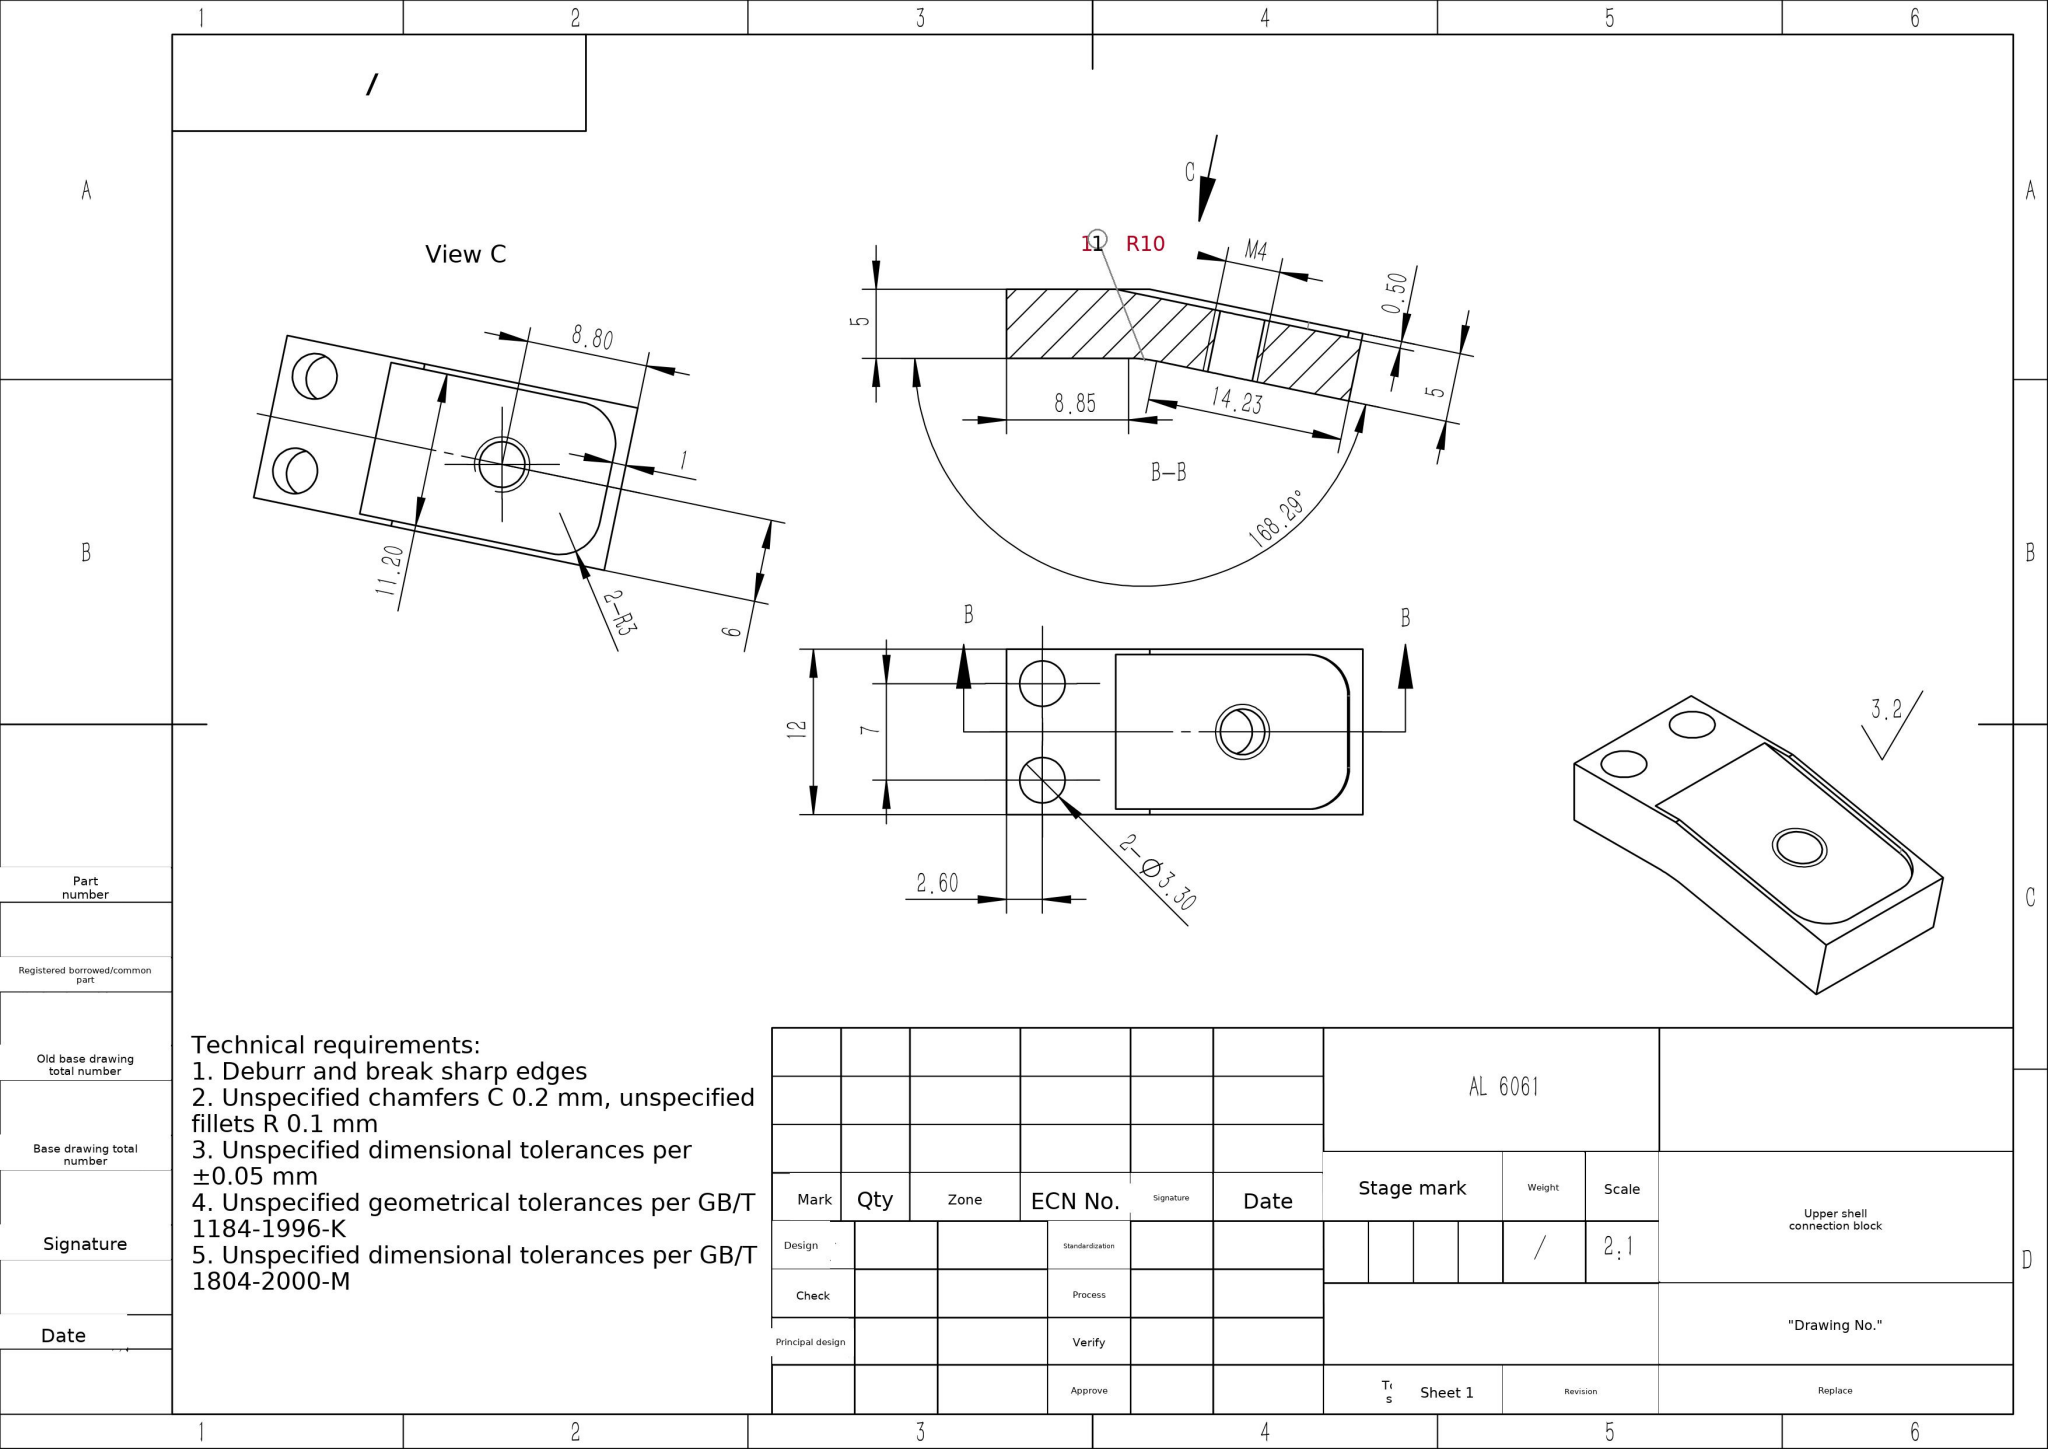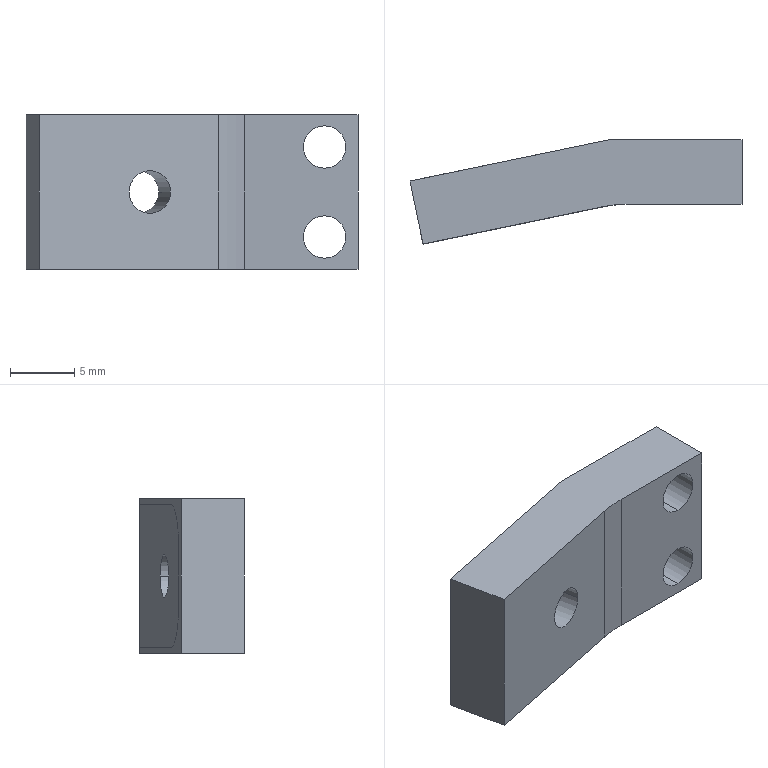Part | SolidWorks | mm | material AL 6061 | 1 solid | 21 faces | box 25.84 x 8.1 x 12 mm | volume 1328 mm3 | plane 12 | cylinder 9 | commonest cylinder face diameters 3.3 x6 6 x2 20 x1
STEP:
#1=CARTESIAN_POINT('',(117.754,277.743,6.));
#2=VERTEX_POINT('',#1);
#3=CARTESIAN_POINT('',(114.523,277.073,6.));
#4=VERTEX_POINT('',#3);
#5=CARTESIAN_POINT('',(116.139,277.408,6.));
#6=DIRECTION('',(-0.203,0.9792,0.));
#7=DIRECTION('',(-0.9792,-0.203,0.));
#8=AXIS2_PLACEMENT_3D('',#5,#6,#7);
#9=CIRCLE('',#8,1.65);
#10=EDGE_CURVE('',#2,#4,#9,.T.);
#11=ORIENTED_EDGE('',*,*,#10,.F.);
#12=CARTESIAN_POINT('',(116.841,282.15,6.));
#13=VERTEX_POINT('',#12);
#14=CARTESIAN_POINT('',(116.841,282.15,6.));
#15=DIRECTION('',(-0.203,0.9792,0.));
#16=VECTOR('',#15,1000.);
#17=LINE('',#14,#16);
#18=EDGE_CURVE('',#2,#13,#17,.T.);
#19=ORIENTED_EDGE('',*,*,#18,.T.);
#20=CARTESIAN_POINT('',(113.609,281.48,6.));
#21=VERTEX_POINT('',#20);
#22=CARTESIAN_POINT('',(115.225,281.815,6.));
#23=DIRECTION('',(-0.203,0.9792,0.));
#24=DIRECTION('',(-0.9792,-0.203,0.));
#25=AXIS2_PLACEMENT_3D('',#22,#23,#24);
#26=CIRCLE('',#25,1.65);
#27=EDGE_CURVE('',#13,#21,#26,.T.);
#28=ORIENTED_EDGE('',*,*,#27,.T.);
#29=CARTESIAN_POINT('',(113.609,281.48,6.));
#30=DIRECTION('',(-0.203,0.9792,0.));
#31=VECTOR('',#30,1000.);
#32=LINE('',#29,#31);
#33=EDGE_CURVE('',#4,#21,#32,.T.);
#34=ORIENTED_EDGE('',*,*,#33,.F.);
#35=EDGE_LOOP('',(#11,#19,#28,#34));
#36=FACE_OUTER_BOUND('',#35,.T.);
#37=CARTESIAN_POINT('',(115.225,281.815,6.));
#38=DIRECTION('',(-0.203,0.9792,0.));
#39=DIRECTION('',(-0.9792,-0.203,0.));
#40=AXIS2_PLACEMENT_3D('',#37,#38,#39);
#41=CYLINDRICAL_SURFACE('',#40,1.65);
#42=ADVANCED_FACE('',(#36),#41,.F.);
#43=CARTESIAN_POINT('',(129.743,278.72,0.85));
#44=VERTEX_POINT('',#43);
#45=CARTESIAN_POINT('',(129.743,278.72,4.15));
#46=VERTEX_POINT('',#45);
#47=CARTESIAN_POINT('',(129.743,278.72,2.5));
#48=DIRECTION('',(0.,1.,0.));
#49=DIRECTION('',(0.,0.,1.));
#50=AXIS2_PLACEMENT_3D('',#47,#48,#49);
#51=CIRCLE('',#50,1.65);
#52=EDGE_CURVE('',#44,#46,#51,.T.);
#53=ORIENTED_EDGE('',*,*,#52,.F.);
#54=CARTESIAN_POINT('',(129.743,283.72,0.85));
#55=VERTEX_POINT('',#54);
#56=CARTESIAN_POINT('',(129.743,267.35,0.85));
#57=DIRECTION('',(0.,1.,0.));
#58=VECTOR('',#57,1000.);
#59=LINE('',#56,#58);
#60=EDGE_CURVE('',#44,#55,#59,.T.);
#61=ORIENTED_EDGE('',*,*,#60,.T.);
#62=CARTESIAN_POINT('',(129.743,283.72,4.15));
#63=VERTEX_POINT('',#62);
#64=CARTESIAN_POINT('',(129.743,283.72,2.5));
#65=DIRECTION('',(0.,1.,0.));
#66=DIRECTION('',(0.,0.,-1.));
#67=AXIS2_PLACEMENT_3D('',#64,#65,#66);
#68=CIRCLE('',#67,1.65);
#69=EDGE_CURVE('',#55,#63,#68,.T.);
#70=ORIENTED_EDGE('',*,*,#69,.T.);
#71=CARTESIAN_POINT('',(129.743,267.35,4.15));
#72=DIRECTION('',(0.,1.,0.));
#73=VECTOR('',#72,1000.);
#74=LINE('',#71,#73);
#75=EDGE_CURVE('',#46,#63,#74,.T.);
#76=ORIENTED_EDGE('',*,*,#75,.F.);
#77=EDGE_LOOP('',(#53,#61,#70,#76));
#78=FACE_OUTER_BOUND('',#77,.T.);
#79=CARTESIAN_POINT('',(129.743,267.35,2.5));
#80=DIRECTION('',(0.,1.,0.));
#81=DIRECTION('',(0.,0.,1.));
#82=AXIS2_PLACEMENT_3D('',#79,#80,#81);
#83=CYLINDRICAL_SURFACE('',#82,1.65);
#84=ADVANCED_FACE('',(#78),#83,.F.);
#85=CARTESIAN_POINT('',(129.743,278.72,7.85));
#86=VERTEX_POINT('',#85);
#87=CARTESIAN_POINT('',(129.743,278.72,11.15));
#88=VERTEX_POINT('',#87);
#89=CARTESIAN_POINT('',(129.743,278.72,9.5));
#90=DIRECTION('',(0.,1.,0.));
#91=DIRECTION('',(0.,0.,1.));
#92=AXIS2_PLACEMENT_3D('',#89,#90,#91);
#93=CIRCLE('',#92,1.65);
#94=EDGE_CURVE('',#86,#88,#93,.T.);
#95=ORIENTED_EDGE('',*,*,#94,.F.);
#96=CARTESIAN_POINT('',(129.743,283.72,7.85));
#97=VERTEX_POINT('',#96);
#98=CARTESIAN_POINT('',(129.743,267.35,7.85));
#99=DIRECTION('',(0.,1.,0.));
#100=VECTOR('',#99,1000.);
#101=LINE('',#98,#100);
#102=EDGE_CURVE('',#86,#97,#101,.T.);
#103=ORIENTED_EDGE('',*,*,#102,.T.);
#104=CARTESIAN_POINT('',(129.743,283.72,11.15));
#105=VERTEX_POINT('',#104);
#106=CARTESIAN_POINT('',(129.743,283.72,9.5));
#107=DIRECTION('',(0.,1.,0.));
#108=DIRECTION('',(0.,0.,-1.));
#109=AXIS2_PLACEMENT_3D('',#106,#107,#108);
#110=CIRCLE('',#109,1.65);
#111=EDGE_CURVE('',#97,#105,#110,.T.);
#112=ORIENTED_EDGE('',*,*,#111,.T.);
#113=CARTESIAN_POINT('',(129.743,267.35,11.15));
#114=DIRECTION('',(0.,1.,0.));
#115=VECTOR('',#114,1000.);
#116=LINE('',#113,#115);
#117=EDGE_CURVE('',#88,#105,#116,.T.);
#118=ORIENTED_EDGE('',*,*,#117,.F.);
#119=EDGE_LOOP('',(#95,#103,#112,#118));
#120=FACE_OUTER_BOUND('',#119,.T.);
#121=CARTESIAN_POINT('',(129.743,267.35,9.5));
#122=DIRECTION('',(0.,1.,0.));
#123=DIRECTION('',(0.,0.,1.));
#124=AXIS2_PLACEMENT_3D('',#121,#122,#123);
#125=CYLINDRICAL_SURFACE('',#124,1.65);
#126=ADVANCED_FACE('',(#120),#125,.F.);
#127=CARTESIAN_POINT('',(115.225,281.815,6.));
#128=DIRECTION('',(-0.203,0.9792,0.));
#129=DIRECTION('',(-0.9792,-0.203,0.));
#130=AXIS2_PLACEMENT_3D('',#127,#128,#129);
#131=CIRCLE('',#130,1.65);
#132=EDGE_CURVE('',#21,#13,#131,.T.);
#133=ORIENTED_EDGE('',*,*,#132,.F.);
#134=ORIENTED_EDGE('',*,*,#27,.F.);
#135=EDGE_LOOP('',(#133,#134));
#136=FACE_BOUND('',#135,.T.);
#137=CARTESIAN_POINT('',(107.588,280.231,8.6));
#138=VERTEX_POINT('',#137);
#139=CARTESIAN_POINT('',(107.588,280.231,3.4));
#140=VERTEX_POINT('',#139);
#141=CARTESIAN_POINT('',(107.588,280.231,0.));
#142=DIRECTION('',(0.,0.,-1.));
#143=VECTOR('',#142,1000.);
#144=LINE('',#141,#143);
#145=EDGE_CURVE('',#138,#140,#144,.T.);
#146=ORIENTED_EDGE('',*,*,#145,.F.);
#147=CARTESIAN_POINT('',(110.525,280.84,11.6));
#148=VERTEX_POINT('',#147);
#149=CARTESIAN_POINT('',(110.525,280.84,8.6));
#150=DIRECTION('',(-0.203,0.9792,0.));
#151=DIRECTION('',(-0.9792,-0.203,0.));
#152=AXIS2_PLACEMENT_3D('',#149,#150,#151);
#153=CIRCLE('',#152,3.);
#154=EDGE_CURVE('',#138,#148,#153,.T.);
#155=ORIENTED_EDGE('',*,*,#154,.T.);
#156=CARTESIAN_POINT('',(124.415,283.72,11.6));
#157=VERTEX_POINT('',#156);
#158=CARTESIAN_POINT('',(129.019,284.675,11.6));
#159=DIRECTION('',(0.9792,0.203,-0.));
#160=VECTOR('',#159,1000.);
#161=LINE('',#158,#160);
#162=EDGE_CURVE('',#148,#157,#161,.T.);
#163=ORIENTED_EDGE('',*,*,#162,.T.);
#164=CARTESIAN_POINT('',(124.415,283.72,0.4));
#165=VERTEX_POINT('',#164);
#166=CARTESIAN_POINT('',(124.415,283.72,16.));
#167=DIRECTION('',(0.,0.,-1.));
#168=VECTOR('',#167,1000.);
#169=LINE('',#166,#168);
#170=EDGE_CURVE('',#157,#165,#169,.T.);
#171=ORIENTED_EDGE('',*,*,#170,.T.);
#172=CARTESIAN_POINT('',(110.525,280.84,0.4));
#173=VERTEX_POINT('',#172);
#174=CARTESIAN_POINT('',(129.019,284.675,0.4));
#175=DIRECTION('',(-0.9792,-0.203,0.));
#176=VECTOR('',#175,1000.);
#177=LINE('',#174,#176);
#178=EDGE_CURVE('',#165,#173,#177,.T.);
#179=ORIENTED_EDGE('',*,*,#178,.T.);
#180=CARTESIAN_POINT('',(110.525,280.84,3.4));
#181=DIRECTION('',(-0.203,0.9792,0.));
#182=DIRECTION('',(-0.9792,-0.203,0.));
#183=AXIS2_PLACEMENT_3D('',#180,#181,#182);
#184=CIRCLE('',#183,3.);
#185=EDGE_CURVE('',#173,#140,#184,.T.);
#186=ORIENTED_EDGE('',*,*,#185,.T.);
#187=EDGE_LOOP('',(#146,#155,#163,#171,#179,#186));
#188=FACE_OUTER_BOUND('',#187,.T.);
#189=CARTESIAN_POINT('',(-51.276,247.291,0.));
#190=DIRECTION('',(-0.203,0.9792,0.));
#191=DIRECTION('',(-0.9792,-0.203,0.));
#192=AXIS2_PLACEMENT_3D('',#189,#190,#191);
#193=PLANE('',#192);
#194=ADVANCED_FACE('',(#136,#188),#193,.T.);
#195=CARTESIAN_POINT('',(110.424,281.33,0.4));
#196=VERTEX_POINT('',#195);
#197=CARTESIAN_POINT('',(121.952,283.72,0.4));
#198=VERTEX_POINT('',#197);
#199=CARTESIAN_POINT('',(106.507,280.517,0.4));
#200=DIRECTION('',(0.9792,0.203,-0.));
#201=VECTOR('',#200,1000.);
#202=LINE('',#199,#201);
#203=EDGE_CURVE('',#196,#198,#202,.T.);
#204=ORIENTED_EDGE('',*,*,#203,.F.);
#205=CARTESIAN_POINT('',(110.525,280.84,0.4));
#206=DIRECTION('',(0.203,-0.9792,0.));
#207=VECTOR('',#206,1000.);
#208=LINE('',#205,#207);
#209=EDGE_CURVE('',#196,#173,#208,.T.);
#210=ORIENTED_EDGE('',*,*,#209,.T.);
#211=ORIENTED_EDGE('',*,*,#178,.F.);
#212=CARTESIAN_POINT('',(121.952,283.72,0.4));
#213=DIRECTION('',(1.,0.,-0.));
#214=VECTOR('',#213,1000.);
#215=LINE('',#212,#214);
#216=EDGE_CURVE('',#198,#165,#215,.T.);
#217=ORIENTED_EDGE('',*,*,#216,.F.);
#218=EDGE_LOOP('',(#204,#210,#211,#217));
#219=FACE_OUTER_BOUND('',#218,.T.);
#220=CARTESIAN_POINT('',(129.019,284.675,0.4));
#221=DIRECTION('',(-0.,-0.,-1.));
#222=DIRECTION('',(-1.,0.,0.));
#223=AXIS2_PLACEMENT_3D('',#220,#221,#222);
#224=PLANE('',#223);
#225=ADVANCED_FACE('',(#219),#224,.F.);
#226=ORIENTED_EDGE('',*,*,#162,.F.);
#227=CARTESIAN_POINT('',(110.424,281.33,11.6));
#228=VERTEX_POINT('',#227);
#229=CARTESIAN_POINT('',(110.424,281.33,11.6));
#230=DIRECTION('',(-0.203,0.9792,-0.));
#231=VECTOR('',#230,1000.);
#232=LINE('',#229,#231);
#233=EDGE_CURVE('',#148,#228,#232,.T.);
#234=ORIENTED_EDGE('',*,*,#233,.T.);
#235=CARTESIAN_POINT('',(121.952,283.72,11.6));
#236=VERTEX_POINT('',#235);
#237=CARTESIAN_POINT('',(106.507,280.517,11.6));
#238=DIRECTION('',(-0.9792,-0.203,0.));
#239=VECTOR('',#238,1000.);
#240=LINE('',#237,#239);
#241=EDGE_CURVE('',#236,#228,#240,.T.);
#242=ORIENTED_EDGE('',*,*,#241,.F.);
#243=CARTESIAN_POINT('',(121.952,283.72,11.6));
#244=DIRECTION('',(-1.,0.,0.));
#245=VECTOR('',#244,1000.);
#246=LINE('',#243,#245);
#247=EDGE_CURVE('',#157,#236,#246,.T.);
#248=ORIENTED_EDGE('',*,*,#247,.F.);
#249=EDGE_LOOP('',(#226,#234,#242,#248));
#250=FACE_OUTER_BOUND('',#249,.T.);
#251=CARTESIAN_POINT('',(129.019,284.675,11.6));
#252=DIRECTION('',(0.,0.,1.));
#253=DIRECTION('',(1.,0.,-0.));
#254=AXIS2_PLACEMENT_3D('',#251,#252,#253);
#255=PLANE('',#254);
#256=ADVANCED_FACE('',(#250),#255,.F.);
#257=CARTESIAN_POINT('',(129.743,278.72,2.5));
#258=DIRECTION('',(0.,1.,0.));
#259=DIRECTION('',(0.,0.,1.));
#260=AXIS2_PLACEMENT_3D('',#257,#258,#259);
#261=CIRCLE('',#260,1.65);
#262=EDGE_CURVE('',#46,#44,#261,.T.);
#263=ORIENTED_EDGE('',*,*,#262,.T.);
#264=ORIENTED_EDGE('',*,*,#52,.T.);
#265=EDGE_LOOP('',(#263,#264));
#266=FACE_BOUND('',#265,.T.);
#267=CARTESIAN_POINT('',(129.743,278.72,9.5));
#268=DIRECTION('',(0.,1.,0.));
#269=DIRECTION('',(0.,0.,1.));
#270=AXIS2_PLACEMENT_3D('',#267,#268,#269);
#271=CIRCLE('',#270,1.65);
#272=EDGE_CURVE('',#88,#86,#271,.T.);
#273=ORIENTED_EDGE('',*,*,#272,.T.);
#274=ORIENTED_EDGE('',*,*,#94,.T.);
#275=EDGE_LOOP('',(#273,#274));
#276=FACE_BOUND('',#275,.T.);
#277=CARTESIAN_POINT('',(123.491,278.72,12.));
#278=VERTEX_POINT('',#277);
#279=CARTESIAN_POINT('',(132.342,278.72,12.));
#280=VERTEX_POINT('',#279);
#281=CARTESIAN_POINT('',(122.465,278.72,12.));
#282=DIRECTION('',(1.,0.,0.));
#283=VECTOR('',#282,1000.);
#284=LINE('',#281,#283);
#285=EDGE_CURVE('',#278,#280,#284,.T.);
#286=ORIENTED_EDGE('',*,*,#285,.F.);
#287=CARTESIAN_POINT('',(123.491,278.72,0.));
#288=VERTEX_POINT('',#287);
#289=CARTESIAN_POINT('',(123.491,278.72,0.));
#290=DIRECTION('',(0.,0.,-1.));
#291=VECTOR('',#290,1000.);
#292=LINE('',#289,#291);
#293=EDGE_CURVE('',#278,#288,#292,.T.);
#294=ORIENTED_EDGE('',*,*,#293,.T.);
#295=CARTESIAN_POINT('',(132.342,278.72,0.));
#296=VERTEX_POINT('',#295);
#297=CARTESIAN_POINT('',(122.465,278.72,0.));
#298=DIRECTION('',(1.,0.,0.));
#299=VECTOR('',#298,1000.);
#300=LINE('',#297,#299);
#301=EDGE_CURVE('',#288,#296,#300,.T.);
#302=ORIENTED_EDGE('',*,*,#301,.T.);
#303=CARTESIAN_POINT('',(132.342,278.72,12.));
#304=DIRECTION('',(0.,0.,-1.));
#305=VECTOR('',#304,1000.);
#306=LINE('',#303,#305);
#307=EDGE_CURVE('',#280,#296,#306,.T.);
#308=ORIENTED_EDGE('',*,*,#307,.F.);
#309=EDGE_LOOP('',(#286,#294,#302,#308));
#310=FACE_OUTER_BOUND('',#309,.T.);
#311=CARTESIAN_POINT('',(122.465,278.72,12.));
#312=DIRECTION('',(0.,1.,0.));
#313=DIRECTION('',(0.,0.,1.));
#314=AXIS2_PLACEMENT_3D('',#311,#312,#313);
#315=PLANE('',#314);
#316=ADVANCED_FACE('',(#266,#276,#310),#315,.F.);
#317=CARTESIAN_POINT('',(132.342,283.72,0.));
#318=VERTEX_POINT('',#317);
#319=CARTESIAN_POINT('',(132.342,278.72,0.));
#320=DIRECTION('',(0.,1.,0.));
#321=VECTOR('',#320,1000.);
#322=LINE('',#319,#321);
#323=EDGE_CURVE('',#296,#318,#322,.T.);
#324=ORIENTED_EDGE('',*,*,#323,.T.);
#325=CARTESIAN_POINT('',(132.342,283.72,12.));
#326=VERTEX_POINT('',#325);
#327=CARTESIAN_POINT('',(132.342,283.72,12.));
#328=DIRECTION('',(0.,0.,1.));
#329=VECTOR('',#328,1000.);
#330=LINE('',#327,#329);
#331=EDGE_CURVE('',#318,#326,#330,.T.);
#332=ORIENTED_EDGE('',*,*,#331,.T.);
#333=CARTESIAN_POINT('',(132.342,278.72,12.));
#334=DIRECTION('',(0.,1.,0.));
#335=VECTOR('',#334,1000.);
#336=LINE('',#333,#335);
#337=EDGE_CURVE('',#280,#326,#336,.T.);
#338=ORIENTED_EDGE('',*,*,#337,.F.);
#339=ORIENTED_EDGE('',*,*,#307,.T.);
#340=EDGE_LOOP('',(#324,#332,#338,#339));
#341=FACE_OUTER_BOUND('',#340,.T.);
#342=CARTESIAN_POINT('',(132.342,278.72,12.));
#343=DIRECTION('',(-1.,0.,0.));
#344=DIRECTION('',(0.,0.,1.));
#345=AXIS2_PLACEMENT_3D('',#342,#343,#344);
#346=PLANE('',#345);
#347=ADVANCED_FACE('',(#341),#346,.F.);
#348=CARTESIAN_POINT('',(121.952,283.72,12.));
#349=VERTEX_POINT('',#348);
#350=CARTESIAN_POINT('',(0.,283.72,12.));
#351=DIRECTION('',(1.,0.,0.));
#352=VECTOR('',#351,1000.);
#353=LINE('',#350,#352);
#354=EDGE_CURVE('',#349,#326,#353,.T.);
#355=ORIENTED_EDGE('',*,*,#354,.F.);
#356=CARTESIAN_POINT('',(106.507,280.517,12.));
#357=VERTEX_POINT('',#356);
#358=CARTESIAN_POINT('',(-51.377,247.78,12.));
#359=DIRECTION('',(0.9792,0.203,0.));
#360=VECTOR('',#359,1000.);
#361=LINE('',#358,#360);
#362=EDGE_CURVE('',#357,#349,#361,.T.);
#363=ORIENTED_EDGE('',*,*,#362,.F.);
#364=CARTESIAN_POINT('',(107.522,275.622,12.));
#365=VERTEX_POINT('',#364);
#366=CARTESIAN_POINT('',(107.522,275.622,12.));
#367=DIRECTION('',(-0.203,0.9792,0.));
#368=VECTOR('',#367,1000.);
#369=LINE('',#366,#368);
#370=EDGE_CURVE('',#365,#357,#369,.T.);
#371=ORIENTED_EDGE('',*,*,#370,.F.);
#372=CARTESIAN_POINT('',(121.461,278.512,12.));
#373=VERTEX_POINT('',#372);
#374=CARTESIAN_POINT('',(-50.362,242.884,12.));
#375=DIRECTION('',(-0.9792,-0.203,0.));
#376=VECTOR('',#375,1000.);
#377=LINE('',#374,#376);
#378=EDGE_CURVE('',#373,#365,#377,.T.);
#379=ORIENTED_EDGE('',*,*,#378,.F.);
#380=CARTESIAN_POINT('',(123.491,268.72,12.));
#381=DIRECTION('',(0.,0.,-1.));
#382=DIRECTION('',(1.,0.,0.));
#383=AXIS2_PLACEMENT_3D('',#380,#381,#382);
#384=CIRCLE('',#383,10.);
#385=EDGE_CURVE('',#373,#278,#384,.T.);
#386=ORIENTED_EDGE('',*,*,#385,.T.);
#387=ORIENTED_EDGE('',*,*,#285,.T.);
#388=ORIENTED_EDGE('',*,*,#337,.T.);
#389=EDGE_LOOP('',(#355,#363,#371,#379,#386,#387,#388));
#390=FACE_OUTER_BOUND('',#389,.T.);
#391=CARTESIAN_POINT('',(0.,0.,12.));
#392=DIRECTION('',(0.,0.,1.));
#393=DIRECTION('',(1.,0.,0.));
#394=AXIS2_PLACEMENT_3D('',#391,#392,#393);
#395=PLANE('',#394);
#396=ADVANCED_FACE('',(#390),#395,.T.);
#397=CARTESIAN_POINT('',(107.522,275.622,0.));
#398=VERTEX_POINT('',#397);
#399=CARTESIAN_POINT('',(106.507,280.517,0.));
#400=VERTEX_POINT('',#399);
#401=CARTESIAN_POINT('',(107.522,275.622,0.));
#402=DIRECTION('',(-0.203,0.9792,0.));
#403=VECTOR('',#402,1000.);
#404=LINE('',#401,#403);
#405=EDGE_CURVE('',#398,#400,#404,.T.);
#406=ORIENTED_EDGE('',*,*,#405,.T.);
#407=CARTESIAN_POINT('',(121.952,283.72,0.));
#408=VERTEX_POINT('',#407);
#409=CARTESIAN_POINT('',(106.507,280.517,0.));
#410=DIRECTION('',(-0.9792,-0.203,0.));
#411=VECTOR('',#410,1000.);
#412=LINE('',#409,#411);
#413=EDGE_CURVE('',#408,#400,#412,.T.);
#414=ORIENTED_EDGE('',*,*,#413,.F.);
#415=CARTESIAN_POINT('',(121.952,283.72,0.));
#416=DIRECTION('',(-1.,0.,0.));
#417=VECTOR('',#416,1000.);
#418=LINE('',#415,#417);
#419=EDGE_CURVE('',#318,#408,#418,.T.);
#420=ORIENTED_EDGE('',*,*,#419,.F.);
#421=ORIENTED_EDGE('',*,*,#323,.F.);
#422=ORIENTED_EDGE('',*,*,#301,.F.);
#423=CARTESIAN_POINT('',(121.461,278.512,0.));
#424=VERTEX_POINT('',#423);
#425=CARTESIAN_POINT('',(123.491,268.72,0.));
#426=DIRECTION('',(0.,0.,1.));
#427=DIRECTION('',(1.,0.,0.));
#428=AXIS2_PLACEMENT_3D('',#425,#426,#427);
#429=CIRCLE('',#428,10.);
#430=EDGE_CURVE('',#288,#424,#429,.T.);
#431=ORIENTED_EDGE('',*,*,#430,.T.);
#432=CARTESIAN_POINT('',(122.465,278.72,0.));
#433=DIRECTION('',(0.9792,0.203,0.));
#434=VECTOR('',#433,1000.);
#435=LINE('',#432,#434);
#436=EDGE_CURVE('',#398,#424,#435,.T.);
#437=ORIENTED_EDGE('',*,*,#436,.F.);
#438=EDGE_LOOP('',(#406,#414,#420,#421,#422,#431,#437));
#439=FACE_OUTER_BOUND('',#438,.T.);
#440=CARTESIAN_POINT('',(0.,0.,0.));
#441=DIRECTION('',(0.,0.,1.));
#442=DIRECTION('',(1.,0.,0.));
#443=AXIS2_PLACEMENT_3D('',#440,#441,#442);
#444=PLANE('',#443);
#445=ADVANCED_FACE('',(#439),#444,.F.);
#446=ORIENTED_EDGE('',*,*,#102,.F.);
#447=ORIENTED_EDGE('',*,*,#272,.F.);
#448=ORIENTED_EDGE('',*,*,#117,.T.);
#449=CARTESIAN_POINT('',(129.743,283.72,9.5));
#450=DIRECTION('',(0.,1.,0.));
#451=DIRECTION('',(0.,0.,-1.));
#452=AXIS2_PLACEMENT_3D('',#449,#450,#451);
#453=CIRCLE('',#452,1.65);
#454=EDGE_CURVE('',#105,#97,#453,.T.);
#455=ORIENTED_EDGE('',*,*,#454,.T.);
#456=EDGE_LOOP('',(#446,#447,#448,#455));
#457=FACE_OUTER_BOUND('',#456,.T.);
#458=CARTESIAN_POINT('',(129.743,267.35,9.5));
#459=DIRECTION('',(0.,1.,0.));
#460=DIRECTION('',(0.,0.,1.));
#461=AXIS2_PLACEMENT_3D('',#458,#459,#460);
#462=CYLINDRICAL_SURFACE('',#461,1.65);
#463=ADVANCED_FACE('',(#457),#462,.F.);
#464=ORIENTED_EDGE('',*,*,#60,.F.);
#465=ORIENTED_EDGE('',*,*,#262,.F.);
#466=ORIENTED_EDGE('',*,*,#75,.T.);
#467=CARTESIAN_POINT('',(129.743,283.72,2.5));
#468=DIRECTION('',(0.,1.,0.));
#469=DIRECTION('',(0.,0.,-1.));
#470=AXIS2_PLACEMENT_3D('',#467,#468,#469);
#471=CIRCLE('',#470,1.65);
#472=EDGE_CURVE('',#63,#55,#471,.T.);
#473=ORIENTED_EDGE('',*,*,#472,.T.);
#474=EDGE_LOOP('',(#464,#465,#466,#473));
#475=FACE_OUTER_BOUND('',#474,.T.);
#476=CARTESIAN_POINT('',(129.743,267.35,2.5));
#477=DIRECTION('',(0.,1.,0.));
#478=DIRECTION('',(0.,0.,1.));
#479=AXIS2_PLACEMENT_3D('',#476,#477,#478);
#480=CYLINDRICAL_SURFACE('',#479,1.65);
#481=ADVANCED_FACE('',(#475),#480,.F.);
#482=CARTESIAN_POINT('',(116.139,277.408,6.));
#483=DIRECTION('',(-0.203,0.9792,0.));
#484=DIRECTION('',(-0.9792,-0.203,0.));
#485=AXIS2_PLACEMENT_3D('',#482,#483,#484);
#486=CIRCLE('',#485,1.65);
#487=EDGE_CURVE('',#4,#2,#486,.T.);
#488=ORIENTED_EDGE('',*,*,#487,.T.);
#489=ORIENTED_EDGE('',*,*,#10,.T.);
#490=EDGE_LOOP('',(#488,#489));
#491=FACE_BOUND('',#490,.T.);
#492=ORIENTED_EDGE('',*,*,#436,.T.);
#493=CARTESIAN_POINT('',(121.461,278.512,12.));
#494=DIRECTION('',(0.,0.,1.));
#495=VECTOR('',#494,1000.);
#496=LINE('',#493,#495);
#497=EDGE_CURVE('',#424,#373,#496,.T.);
#498=ORIENTED_EDGE('',*,*,#497,.T.);
#499=ORIENTED_EDGE('',*,*,#378,.T.);
#500=CARTESIAN_POINT('',(107.522,275.622,12.));
#501=DIRECTION('',(0.,0.,1.));
#502=VECTOR('',#501,1000.);
#503=LINE('',#500,#502);
#504=EDGE_CURVE('',#398,#365,#503,.T.);
#505=ORIENTED_EDGE('',*,*,#504,.F.);
#506=EDGE_LOOP('',(#492,#498,#499,#505));
#507=FACE_OUTER_BOUND('',#506,.T.);
#508=CARTESIAN_POINT('',(122.465,278.72,16.));
#509=DIRECTION('',(-0.203,0.9792,0.));
#510=DIRECTION('',(-0.9792,-0.203,0.));
#511=AXIS2_PLACEMENT_3D('',#508,#509,#510);
#512=PLANE('',#511);
#513=ADVANCED_FACE('',(#491,#507),#512,.F.);
#514=CARTESIAN_POINT('',(106.507,280.517,19.679));
#515=DIRECTION('',(0.,0.,1.));
#516=VECTOR('',#515,1000.);
#517=LINE('',#514,#516);
#518=EDGE_CURVE('',#400,#357,#517,.T.);
#519=ORIENTED_EDGE('',*,*,#518,.F.);
#520=ORIENTED_EDGE('',*,*,#405,.F.);
#521=ORIENTED_EDGE('',*,*,#504,.T.);
#522=ORIENTED_EDGE('',*,*,#370,.T.);
#523=EDGE_LOOP('',(#519,#520,#521,#522));
#524=FACE_OUTER_BOUND('',#523,.T.);
#525=CARTESIAN_POINT('',(107.522,275.622,19.679));
#526=DIRECTION('',(-0.9792,-0.203,0.));
#527=DIRECTION('',(0.203,-0.9792,0.));
#528=AXIS2_PLACEMENT_3D('',#525,#526,#527);
#529=PLANE('',#528);
#530=ADVANCED_FACE('',(#524),#529,.T.);
#531=CARTESIAN_POINT('',(121.952,283.72,16.));
#532=DIRECTION('',(0.,0.,-1.));
#533=VECTOR('',#532,1000.);
#534=LINE('',#531,#533);
#535=EDGE_CURVE('',#198,#408,#534,.T.);
#536=ORIENTED_EDGE('',*,*,#535,.F.);
#537=ORIENTED_EDGE('',*,*,#216,.T.);
#538=ORIENTED_EDGE('',*,*,#170,.F.);
#539=ORIENTED_EDGE('',*,*,#247,.T.);
#540=CARTESIAN_POINT('',(121.952,283.72,16.));
#541=DIRECTION('',(0.,0.,-1.));
#542=VECTOR('',#541,1000.);
#543=LINE('',#540,#542);
#544=EDGE_CURVE('',#349,#236,#543,.T.);
#545=ORIENTED_EDGE('',*,*,#544,.F.);
#546=ORIENTED_EDGE('',*,*,#354,.T.);
#547=ORIENTED_EDGE('',*,*,#331,.F.);
#548=ORIENTED_EDGE('',*,*,#419,.T.);
#549=EDGE_LOOP('',(#536,#537,#538,#539,#545,#546,#547,#548));
#550=FACE_OUTER_BOUND('',#549,.T.);
#551=ORIENTED_EDGE('',*,*,#472,.F.);
#552=ORIENTED_EDGE('',*,*,#69,.F.);
#553=EDGE_LOOP('',(#551,#552));
#554=FACE_BOUND('',#553,.T.);
#555=ORIENTED_EDGE('',*,*,#454,.F.);
#556=ORIENTED_EDGE('',*,*,#111,.F.);
#557=EDGE_LOOP('',(#555,#556));
#558=FACE_BOUND('',#557,.T.);
#559=CARTESIAN_POINT('',(121.952,283.72,16.));
#560=DIRECTION('',(0.,-1.,0.));
#561=DIRECTION('',(0.,0.,-1.));
#562=AXIS2_PLACEMENT_3D('',#559,#560,#561);
#563=PLANE('',#562);
#564=ADVANCED_FACE('',(#550,#554,#558),#563,.F.);
#565=ORIENTED_EDGE('',*,*,#362,.T.);
#566=ORIENTED_EDGE('',*,*,#544,.T.);
#567=ORIENTED_EDGE('',*,*,#241,.T.);
#568=CARTESIAN_POINT('',(107.486,280.72,8.6));
#569=VERTEX_POINT('',#568);
#570=CARTESIAN_POINT('',(110.424,281.33,8.6));
#571=DIRECTION('',(0.203,-0.9792,0.));
#572=DIRECTION('',(0.9792,0.203,0.));
#573=AXIS2_PLACEMENT_3D('',#570,#571,#572);
#574=CIRCLE('',#573,3.);
#575=EDGE_CURVE('',#228,#569,#574,.T.);
#576=ORIENTED_EDGE('',*,*,#575,.T.);
#577=CARTESIAN_POINT('',(107.486,280.72,3.4));
#578=VERTEX_POINT('',#577);
#579=CARTESIAN_POINT('',(107.486,280.72,0.));
#580=DIRECTION('',(0.,0.,-1.));
#581=VECTOR('',#580,1000.);
#582=LINE('',#579,#581);
#583=EDGE_CURVE('',#569,#578,#582,.T.);
#584=ORIENTED_EDGE('',*,*,#583,.T.);
#585=CARTESIAN_POINT('',(110.424,281.33,3.4));
#586=DIRECTION('',(0.203,-0.9792,0.));
#587=DIRECTION('',(0.9792,0.203,0.));
#588=AXIS2_PLACEMENT_3D('',#585,#586,#587);
#589=CIRCLE('',#588,3.);
#590=EDGE_CURVE('',#578,#196,#589,.T.);
#591=ORIENTED_EDGE('',*,*,#590,.T.);
#592=ORIENTED_EDGE('',*,*,#203,.T.);
#593=ORIENTED_EDGE('',*,*,#535,.T.);
#594=ORIENTED_EDGE('',*,*,#413,.T.);
#595=ORIENTED_EDGE('',*,*,#518,.T.);
#596=EDGE_LOOP('',(#565,#566,#567,#576,#584,#591,#592,#593,#594,#595));
#597=FACE_OUTER_BOUND('',#596,.T.);
#598=CARTESIAN_POINT('',(106.507,280.517,16.));
#599=DIRECTION('',(0.203,-0.9792,0.));
#600=DIRECTION('',(0.9792,0.203,0.));
#601=AXIS2_PLACEMENT_3D('',#598,#599,#600);
#602=PLANE('',#601);
#603=ADVANCED_FACE('',(#597),#602,.F.);
#604=ORIENTED_EDGE('',*,*,#18,.F.);
#605=ORIENTED_EDGE('',*,*,#487,.F.);
#606=ORIENTED_EDGE('',*,*,#33,.T.);
#607=ORIENTED_EDGE('',*,*,#132,.T.);
#608=EDGE_LOOP('',(#604,#605,#606,#607));
#609=FACE_OUTER_BOUND('',#608,.T.);
#610=CARTESIAN_POINT('',(115.225,281.815,6.));
#611=DIRECTION('',(-0.203,0.9792,0.));
#612=DIRECTION('',(-0.9792,-0.203,0.));
#613=AXIS2_PLACEMENT_3D('',#610,#611,#612);
#614=CYLINDRICAL_SURFACE('',#613,1.65);
#615=ADVANCED_FACE('',(#609),#614,.F.);
#616=ORIENTED_EDGE('',*,*,#583,.F.);
#617=CARTESIAN_POINT('',(107.588,280.231,8.6));
#618=DIRECTION('',(0.203,-0.9792,0.));
#619=VECTOR('',#618,1000.);
#620=LINE('',#617,#619);
#621=EDGE_CURVE('',#569,#138,#620,.T.);
#622=ORIENTED_EDGE('',*,*,#621,.T.);
#623=ORIENTED_EDGE('',*,*,#145,.T.);
#624=CARTESIAN_POINT('',(107.486,280.72,3.4));
#625=DIRECTION('',(-0.203,0.9792,-0.));
#626=VECTOR('',#625,1000.);
#627=LINE('',#624,#626);
#628=EDGE_CURVE('',#140,#578,#627,.T.);
#629=ORIENTED_EDGE('',*,*,#628,.T.);
#630=EDGE_LOOP('',(#616,#622,#623,#629));
#631=FACE_OUTER_BOUND('',#630,.T.);
#632=CARTESIAN_POINT('',(107.486,280.72,0.));
#633=DIRECTION('',(-0.9792,-0.203,0.));
#634=DIRECTION('',(0.203,-0.9792,0.));
#635=AXIS2_PLACEMENT_3D('',#632,#633,#634);
#636=PLANE('',#635);
#637=ADVANCED_FACE('',(#631),#636,.F.);
#638=ORIENTED_EDGE('',*,*,#575,.F.);
#639=ORIENTED_EDGE('',*,*,#233,.F.);
#640=ORIENTED_EDGE('',*,*,#154,.F.);
#641=ORIENTED_EDGE('',*,*,#621,.F.);
#642=EDGE_LOOP('',(#638,#639,#640,#641));
#643=FACE_OUTER_BOUND('',#642,.T.);
#644=CARTESIAN_POINT('',(110.424,281.33,8.6));
#645=DIRECTION('',(-0.203,0.9792,-0.));
#646=DIRECTION('',(-0.9792,-0.203,0.));
#647=AXIS2_PLACEMENT_3D('',#644,#645,#646);
#648=CYLINDRICAL_SURFACE('',#647,3.);
#649=ADVANCED_FACE('',(#643),#648,.F.);
#650=ORIENTED_EDGE('',*,*,#185,.F.);
#651=ORIENTED_EDGE('',*,*,#209,.F.);
#652=ORIENTED_EDGE('',*,*,#590,.F.);
#653=ORIENTED_EDGE('',*,*,#628,.F.);
#654=EDGE_LOOP('',(#650,#651,#652,#653));
#655=FACE_OUTER_BOUND('',#654,.T.);
#656=CARTESIAN_POINT('',(110.424,281.33,3.4));
#657=DIRECTION('',(0.203,-0.9792,0.));
#658=DIRECTION('',(0.9792,0.203,0.));
#659=AXIS2_PLACEMENT_3D('',#656,#657,#658);
#660=CYLINDRICAL_SURFACE('',#659,3.);
#661=ADVANCED_FACE('',(#655),#660,.F.);
#662=ORIENTED_EDGE('',*,*,#385,.F.);
#663=ORIENTED_EDGE('',*,*,#497,.F.);
#664=ORIENTED_EDGE('',*,*,#430,.F.);
#665=ORIENTED_EDGE('',*,*,#293,.F.);
#666=EDGE_LOOP('',(#662,#663,#664,#665));
#667=FACE_OUTER_BOUND('',#666,.T.);
#668=CARTESIAN_POINT('',(123.491,268.72,12.));
#669=DIRECTION('',(0.,0.,1.));
#670=DIRECTION('',(1.,0.,0.));
#671=AXIS2_PLACEMENT_3D('',#668,#669,#670);
#672=CYLINDRICAL_SURFACE('',#671,10.);
#673=ADVANCED_FACE('',(#667),#672,.F.);
#674=CLOSED_SHELL('',(#42,#84,#126,#194,#225,#256,#316,#347,#396,#445,#463,#481,#513,#530,#564,#603,#615,#637,#649,#661,#673));
#675=MANIFOLD_SOLID_BREP('',#674);
#676=CARTESIAN_POINT('',(0.,0.,0.));
#677=DIRECTION('',(0.,0.,1.));
#678=DIRECTION('',(1.,0.,0.));
#679=AXIS2_PLACEMENT_3D('',#676,#677,#678);
#680=(LENGTH_UNIT()NAMED_UNIT(*)SI_UNIT(.MILLI.,.METRE.));
#681=UNCERTAINTY_MEASURE_WITH_UNIT(LENGTH_MEASURE(0.00001),#680,'','');
#682=(NAMED_UNIT(*)PLANE_ANGLE_UNIT()SI_UNIT($,.RADIAN.));
#683=(NAMED_UNIT(*)SI_UNIT($,.STERADIAN.)SOLID_ANGLE_UNIT());
#684=(GEOMETRIC_REPRESENTATION_CONTEXT(3)GLOBAL_UNCERTAINTY_ASSIGNED_CONTEXT((#681))GLOBAL_UNIT_ASSIGNED_CONTEXT((#680,#682,#683))REPRESENTATION_CONTEXT('',''));
#685=ADVANCED_BREP_SHAPE_REPRESENTATION('',(#675,#679),#684);